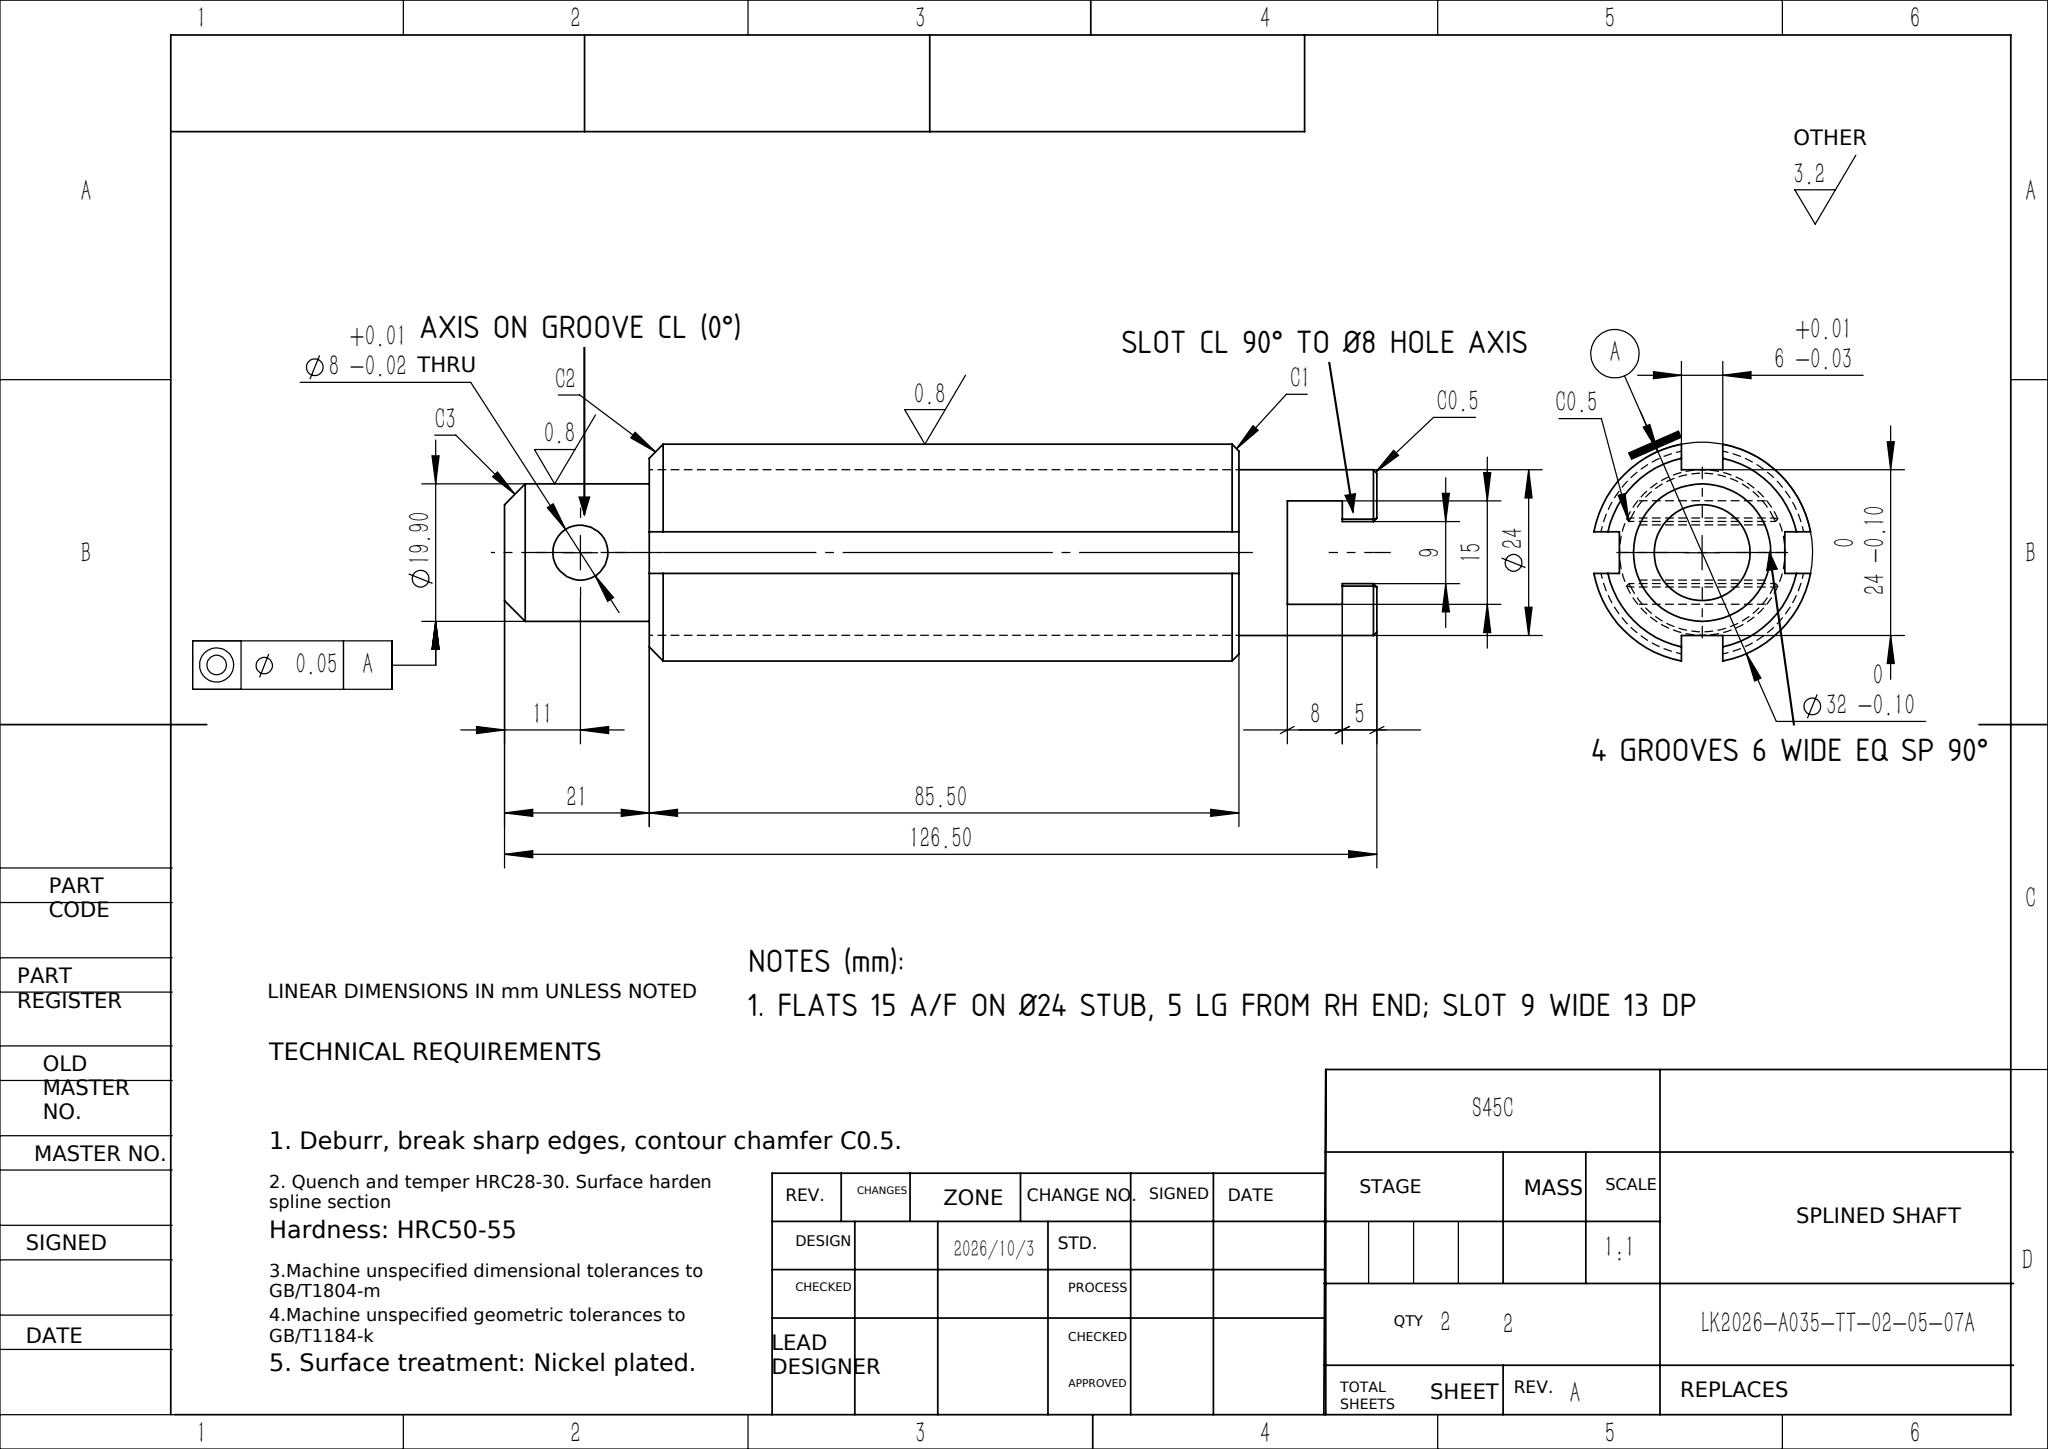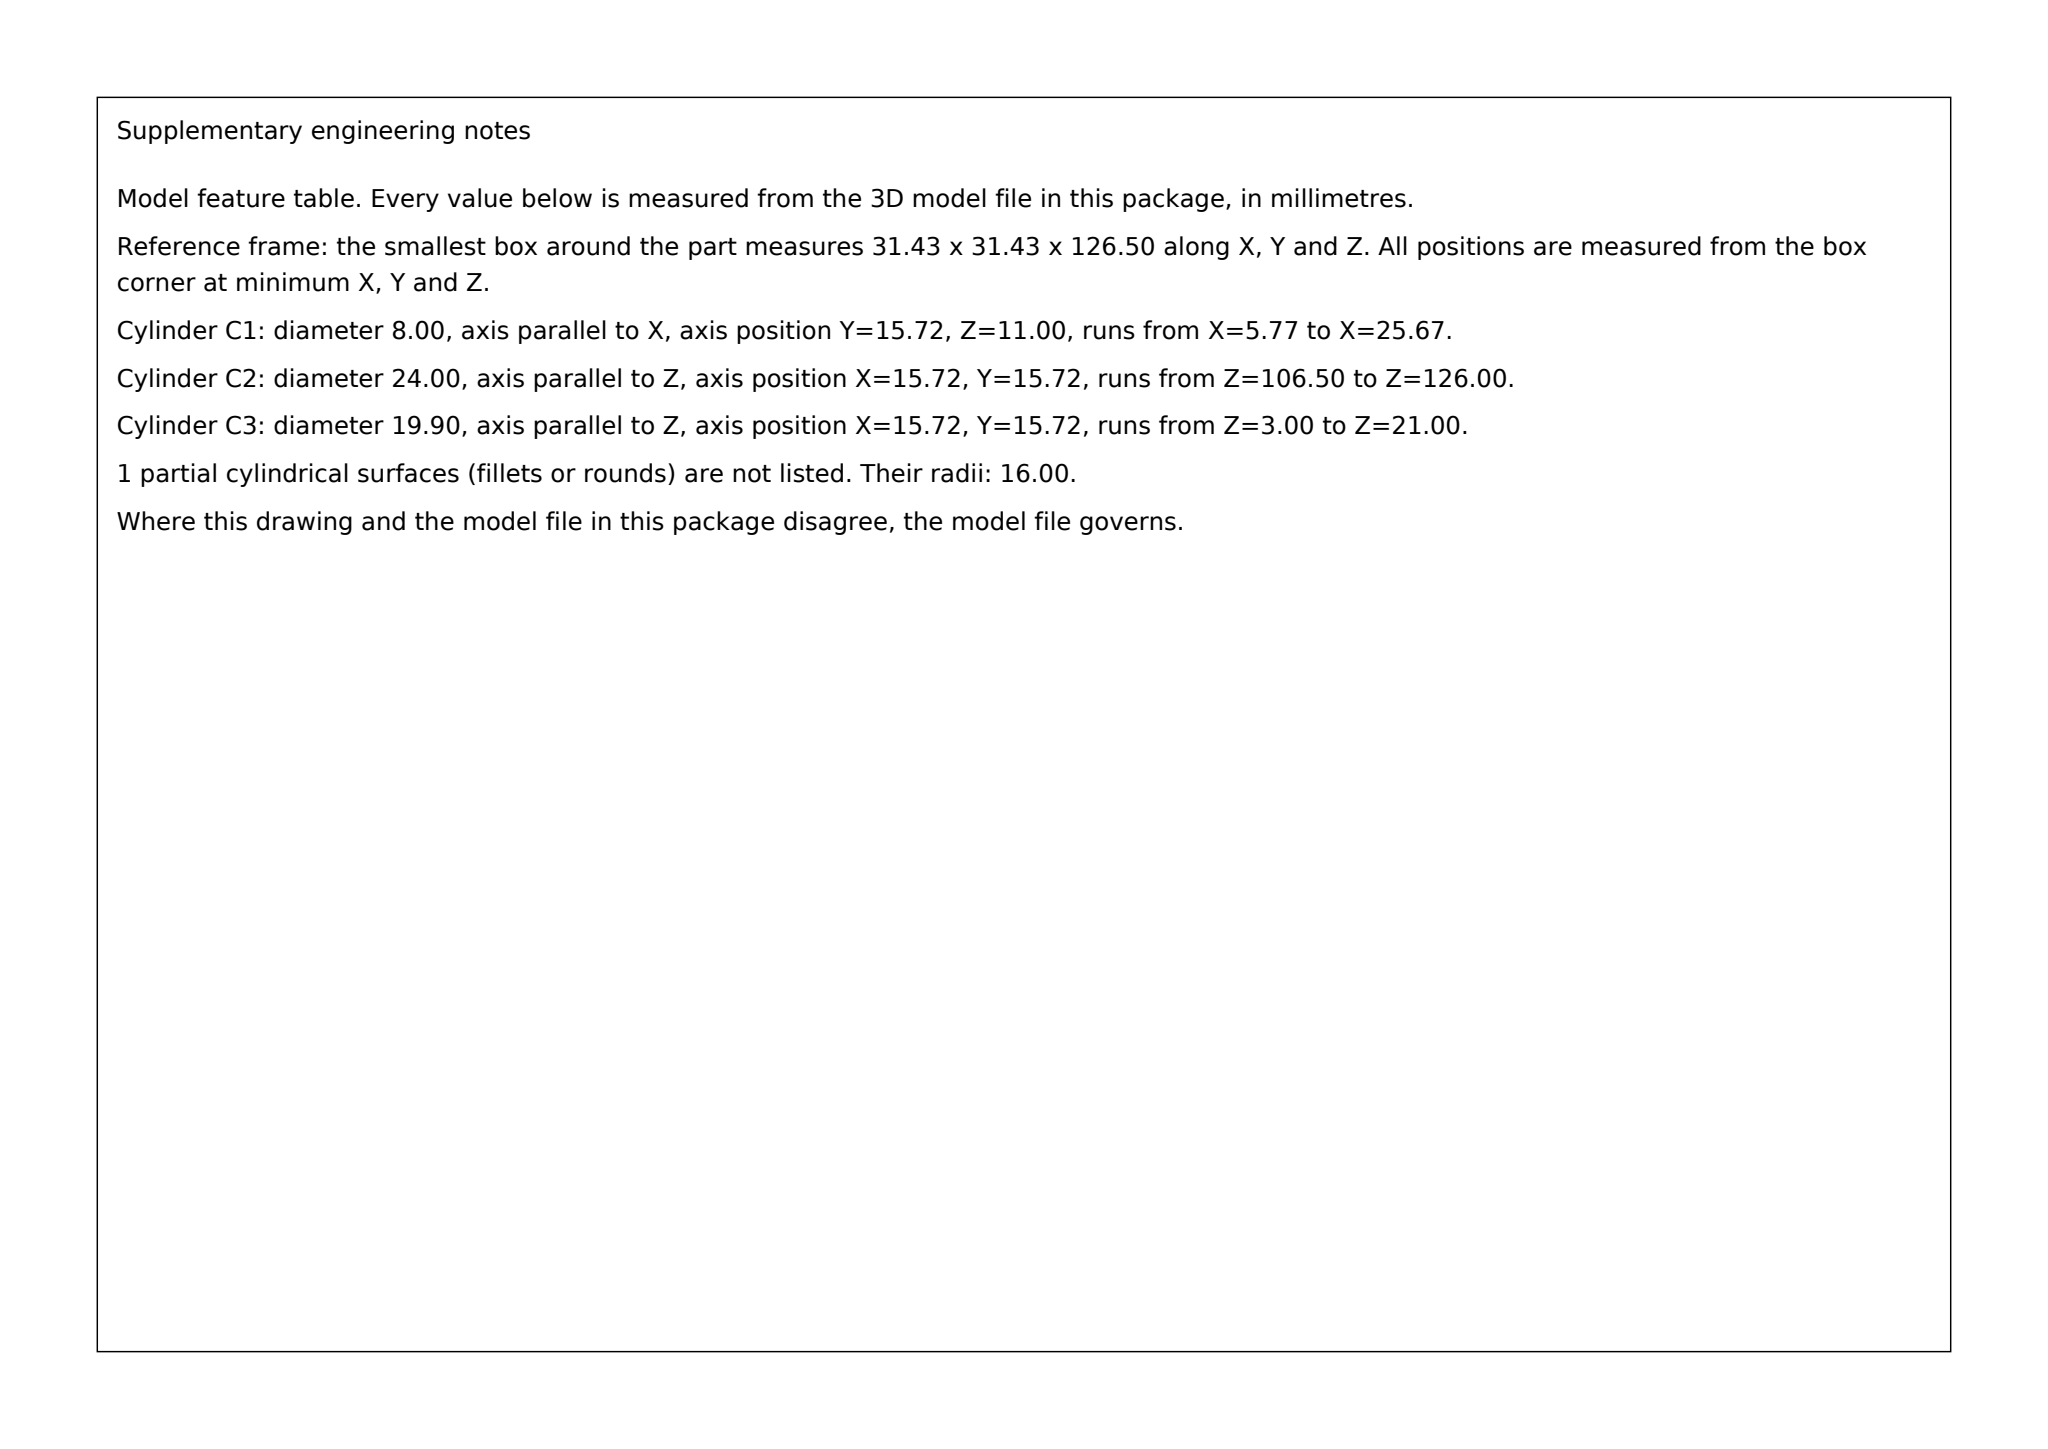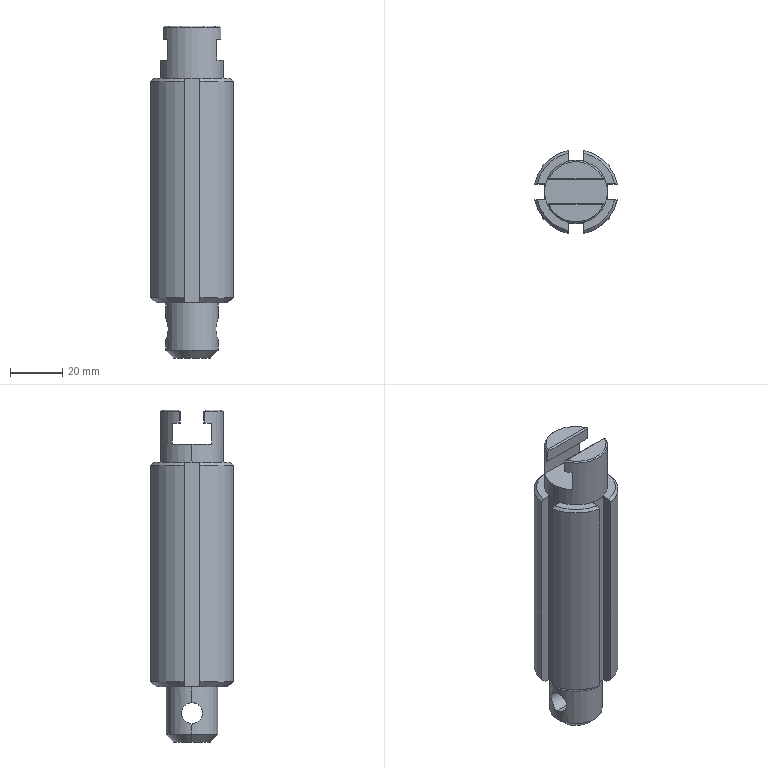Part | SolidWorks | mm | material S45C | 1 solid | 59 faces | box 31.43 x 31.43 x 126.5 mm | volume 71166 mm3 | plane 37 | cone 12 | cylinder 10 | commonest cylinder face diameters 32 x4 8 x2 19.9 x2 24 x2
Drawing notes:
SPLINE: 4 GROOVES 6 WIDE EQ SP 90 DEG ON Ø32 | from the solid: Axis planes x=12.72/18.72 and y=12.72/18.72 (6 wide, centred on axis 15.72) give 4 slots at 90 deg; Ø32 cyl, groove bottoms at 3.72 & 27.72 = 24 across
Ø8 CROSS HOLE AXIS ON SPLINE GROOVE CL - CLOCKED 0 DEG | from the solid: Ø8 hole axis along X at y=15.72, z=11.0; spline groove flanks at y=12.72/18.72 (6 wide) centre grooves on ±X, hole axis coincident with groove CL
RH END FLATS/SLOT CLOCKED 90 DEG TO Ø8 HOLE AXIS, ON GROOVE CL | from the solid: End faces at y=8.22/23.22 (15 wide) and y=11.22/20.22 (9 wide) all normal to Y, symm about y=15.72; hole axis along X; spline grooves also on ±Y
FLATS 15 A/F ON Ø24 STUB, 5 LG FROM RH END; SLOT 9 WIDE 13 DP | from the solid: y-planes 8.22 & 23.22 = 15 A/F, end walls z=121.5, part end z=126.5 -> 5 lg; y-planes 11.22 & 20.22 = 9 wide, end wall z=113.5 -> 13 dp; Ø24 stub z=106.5-126.5